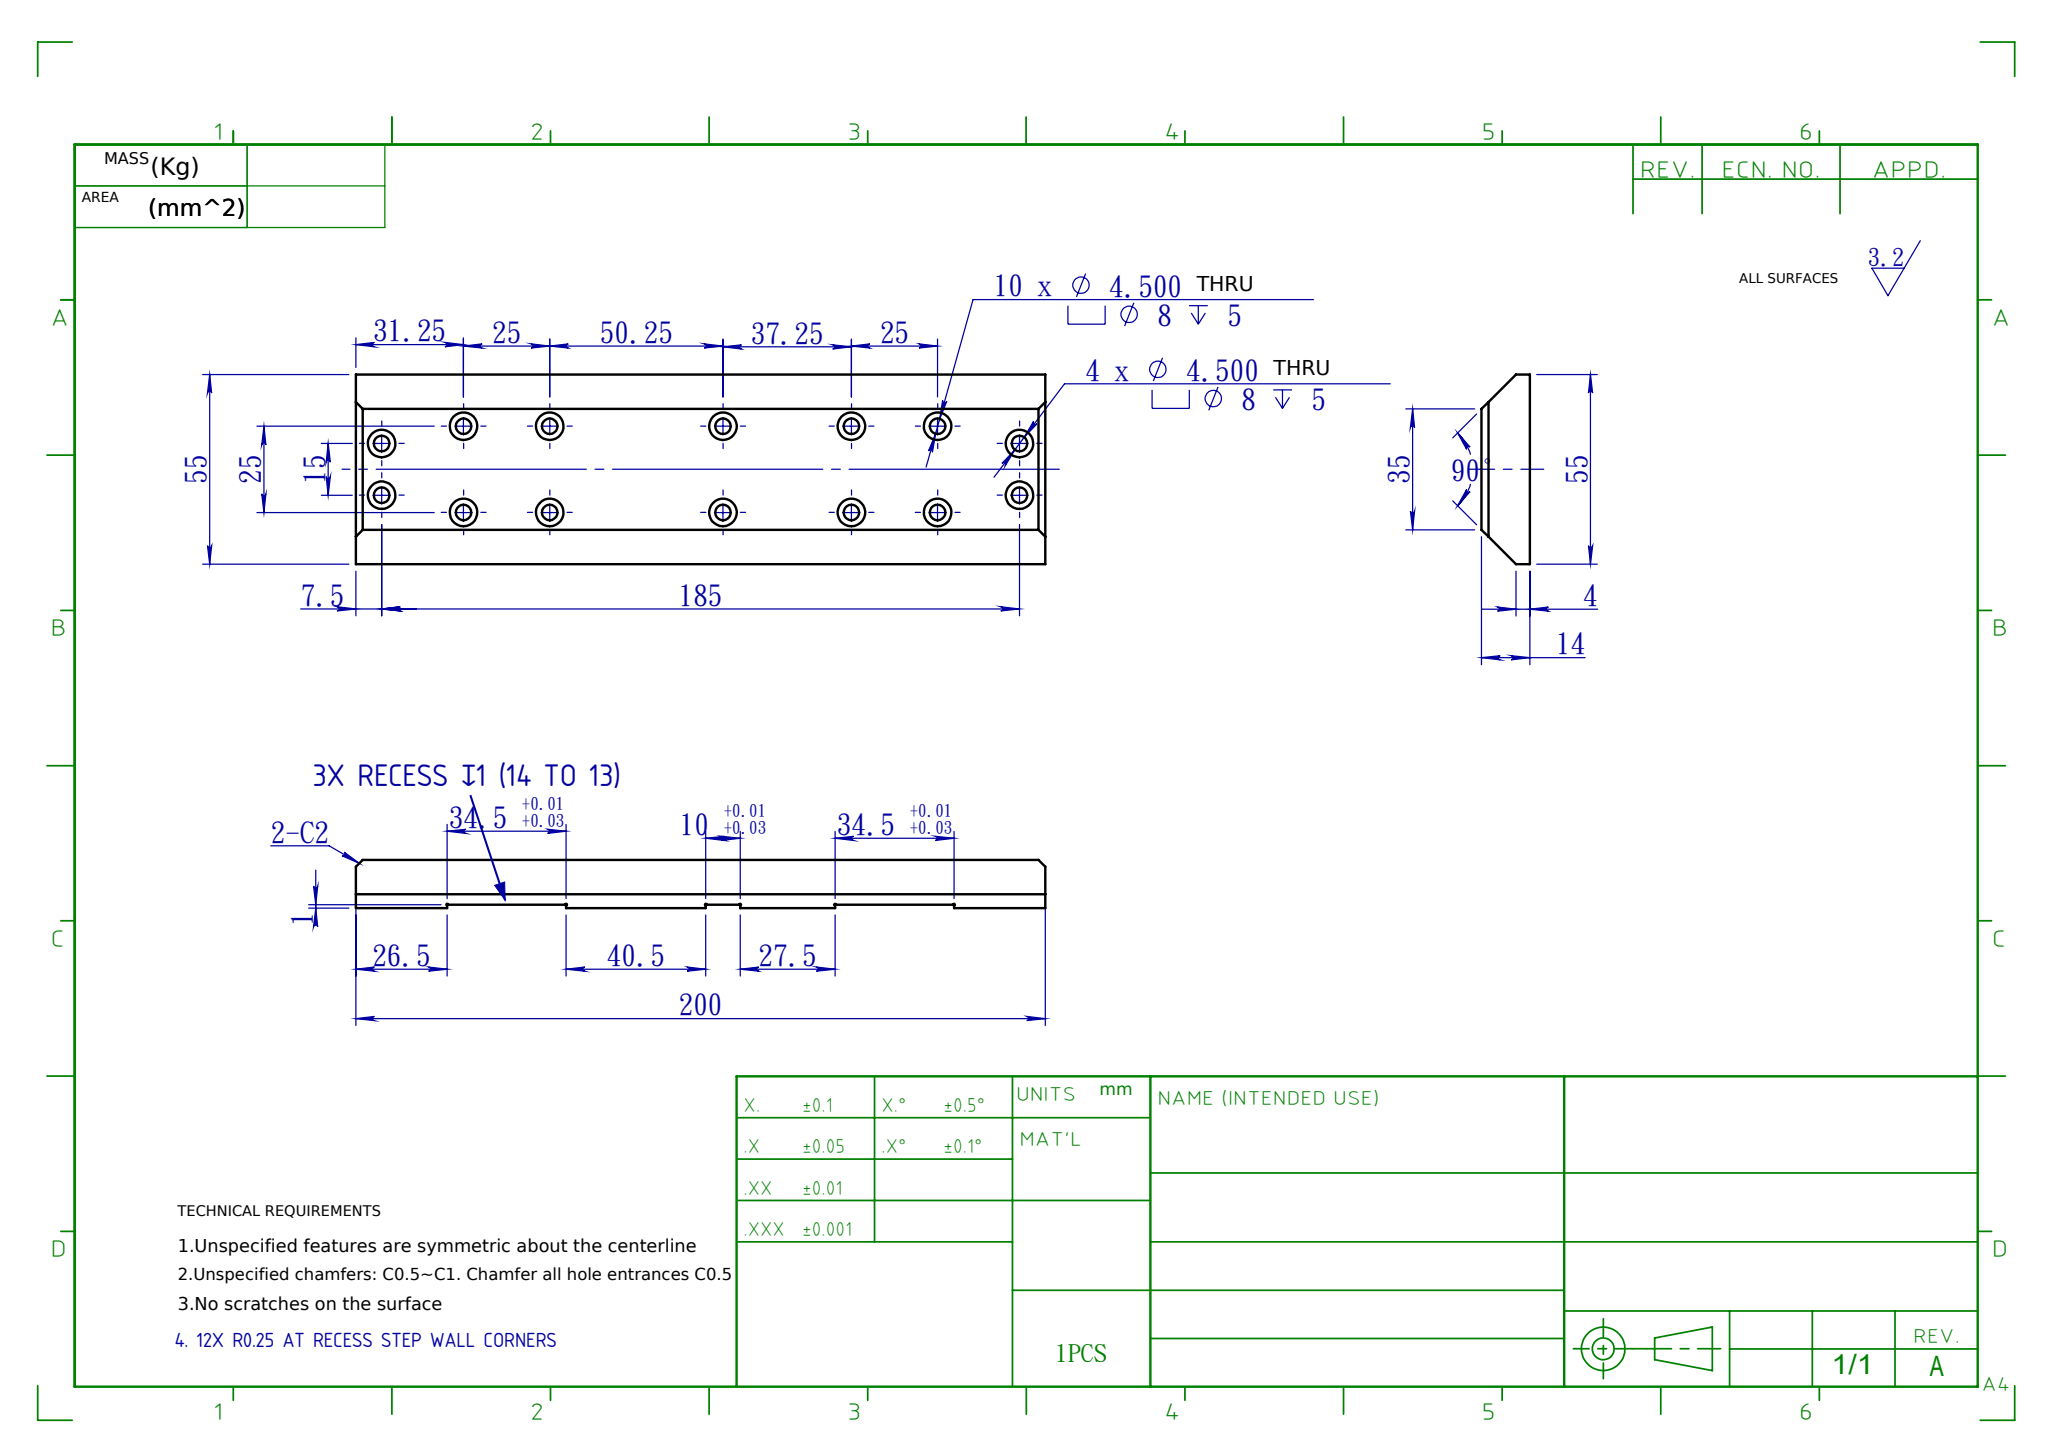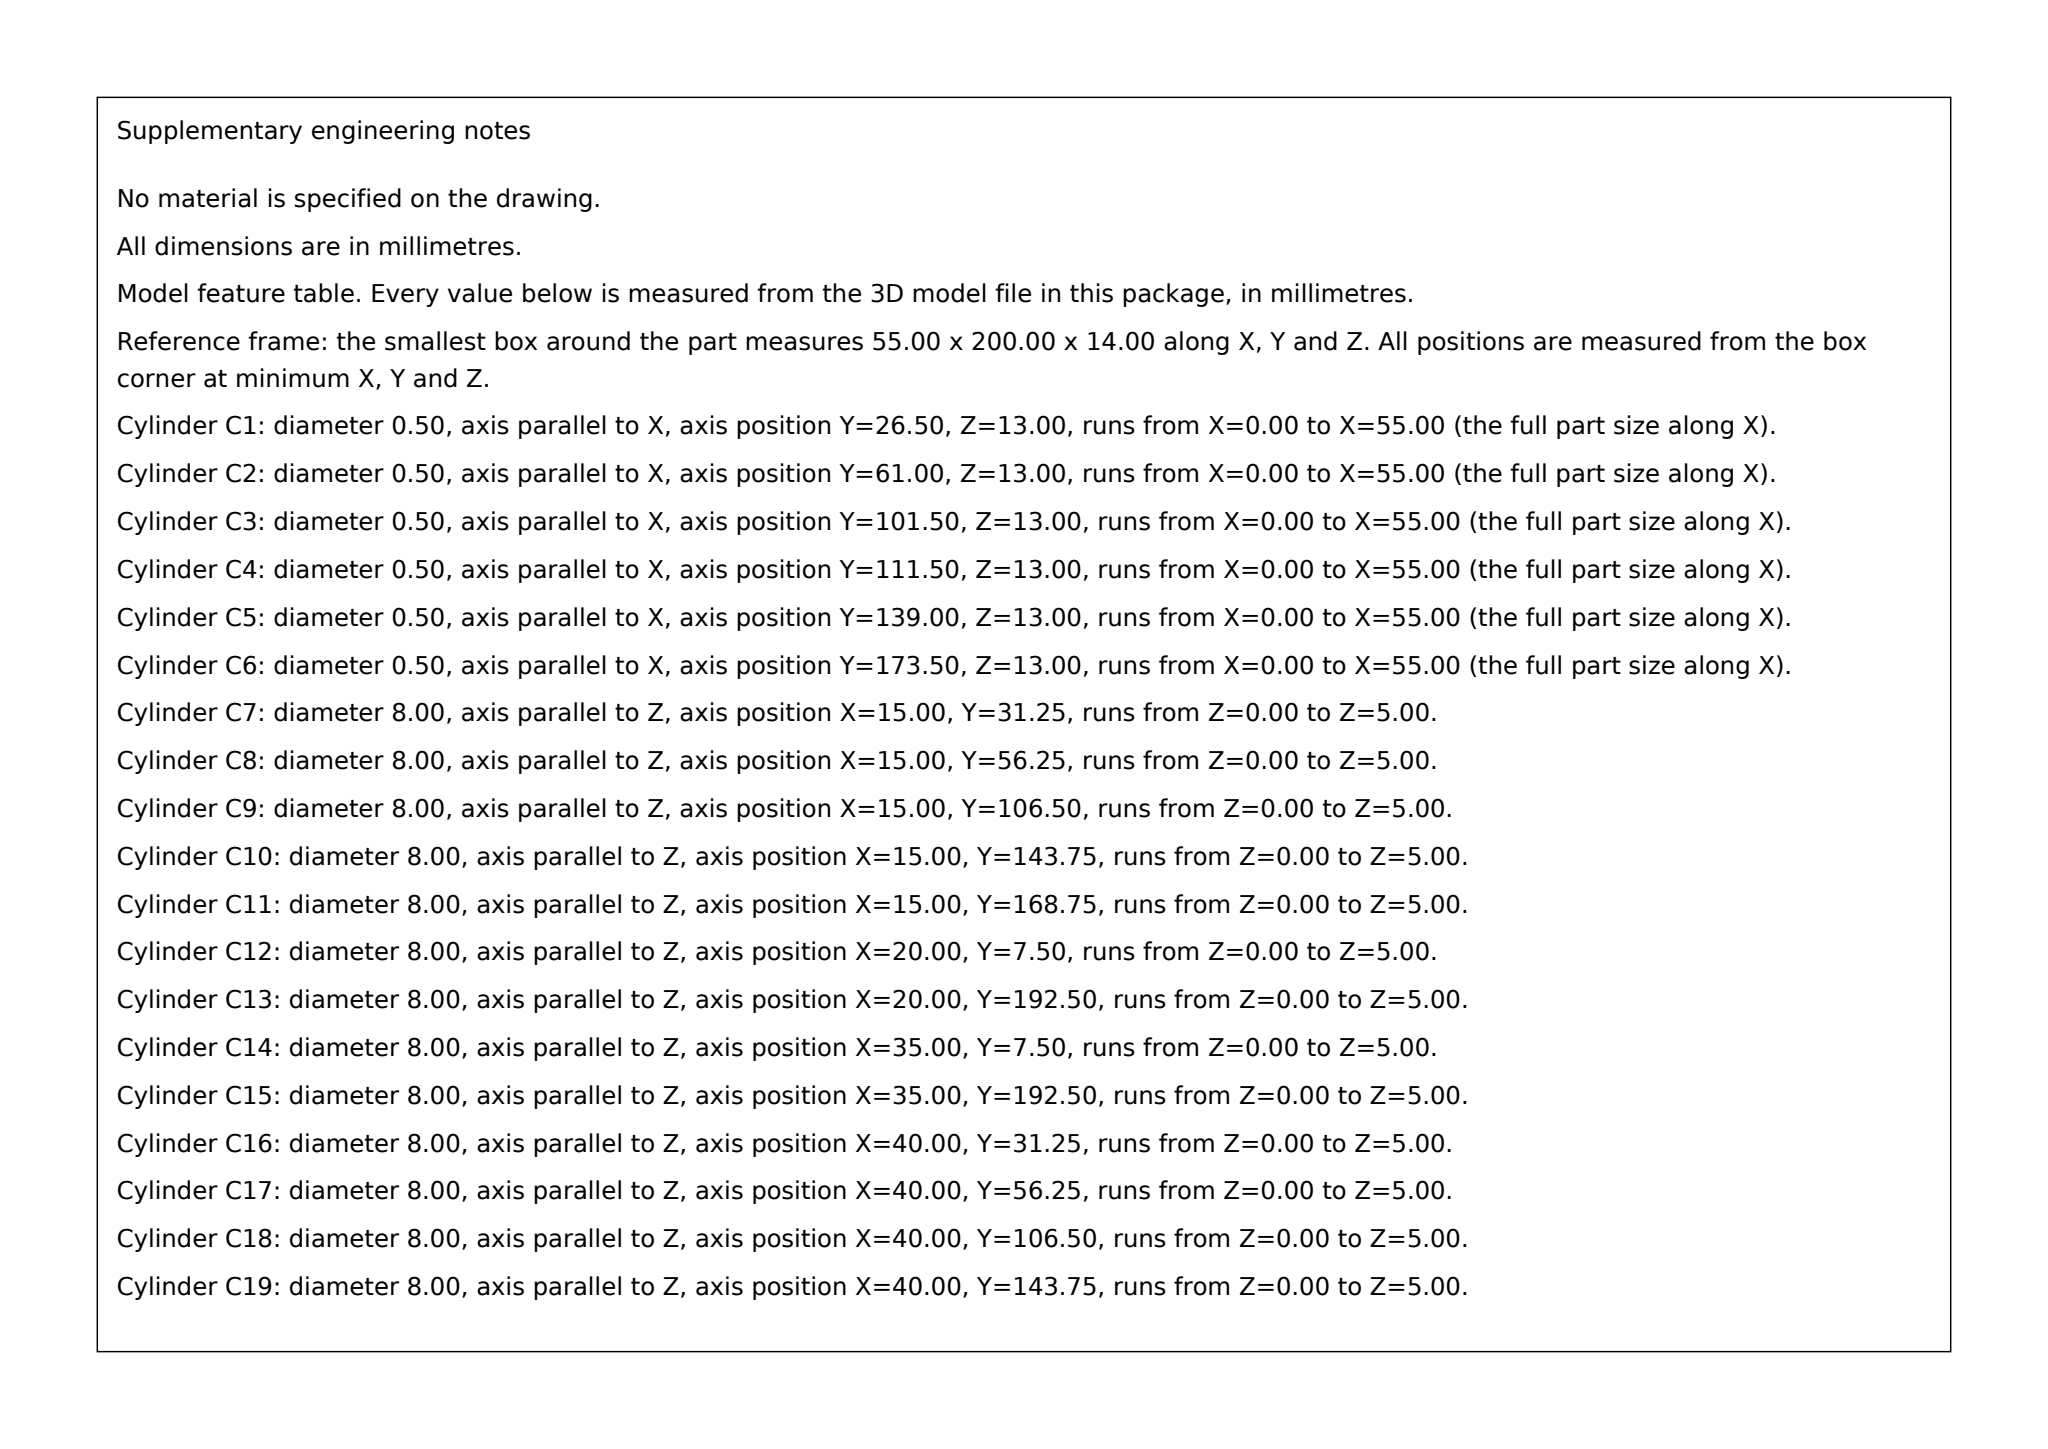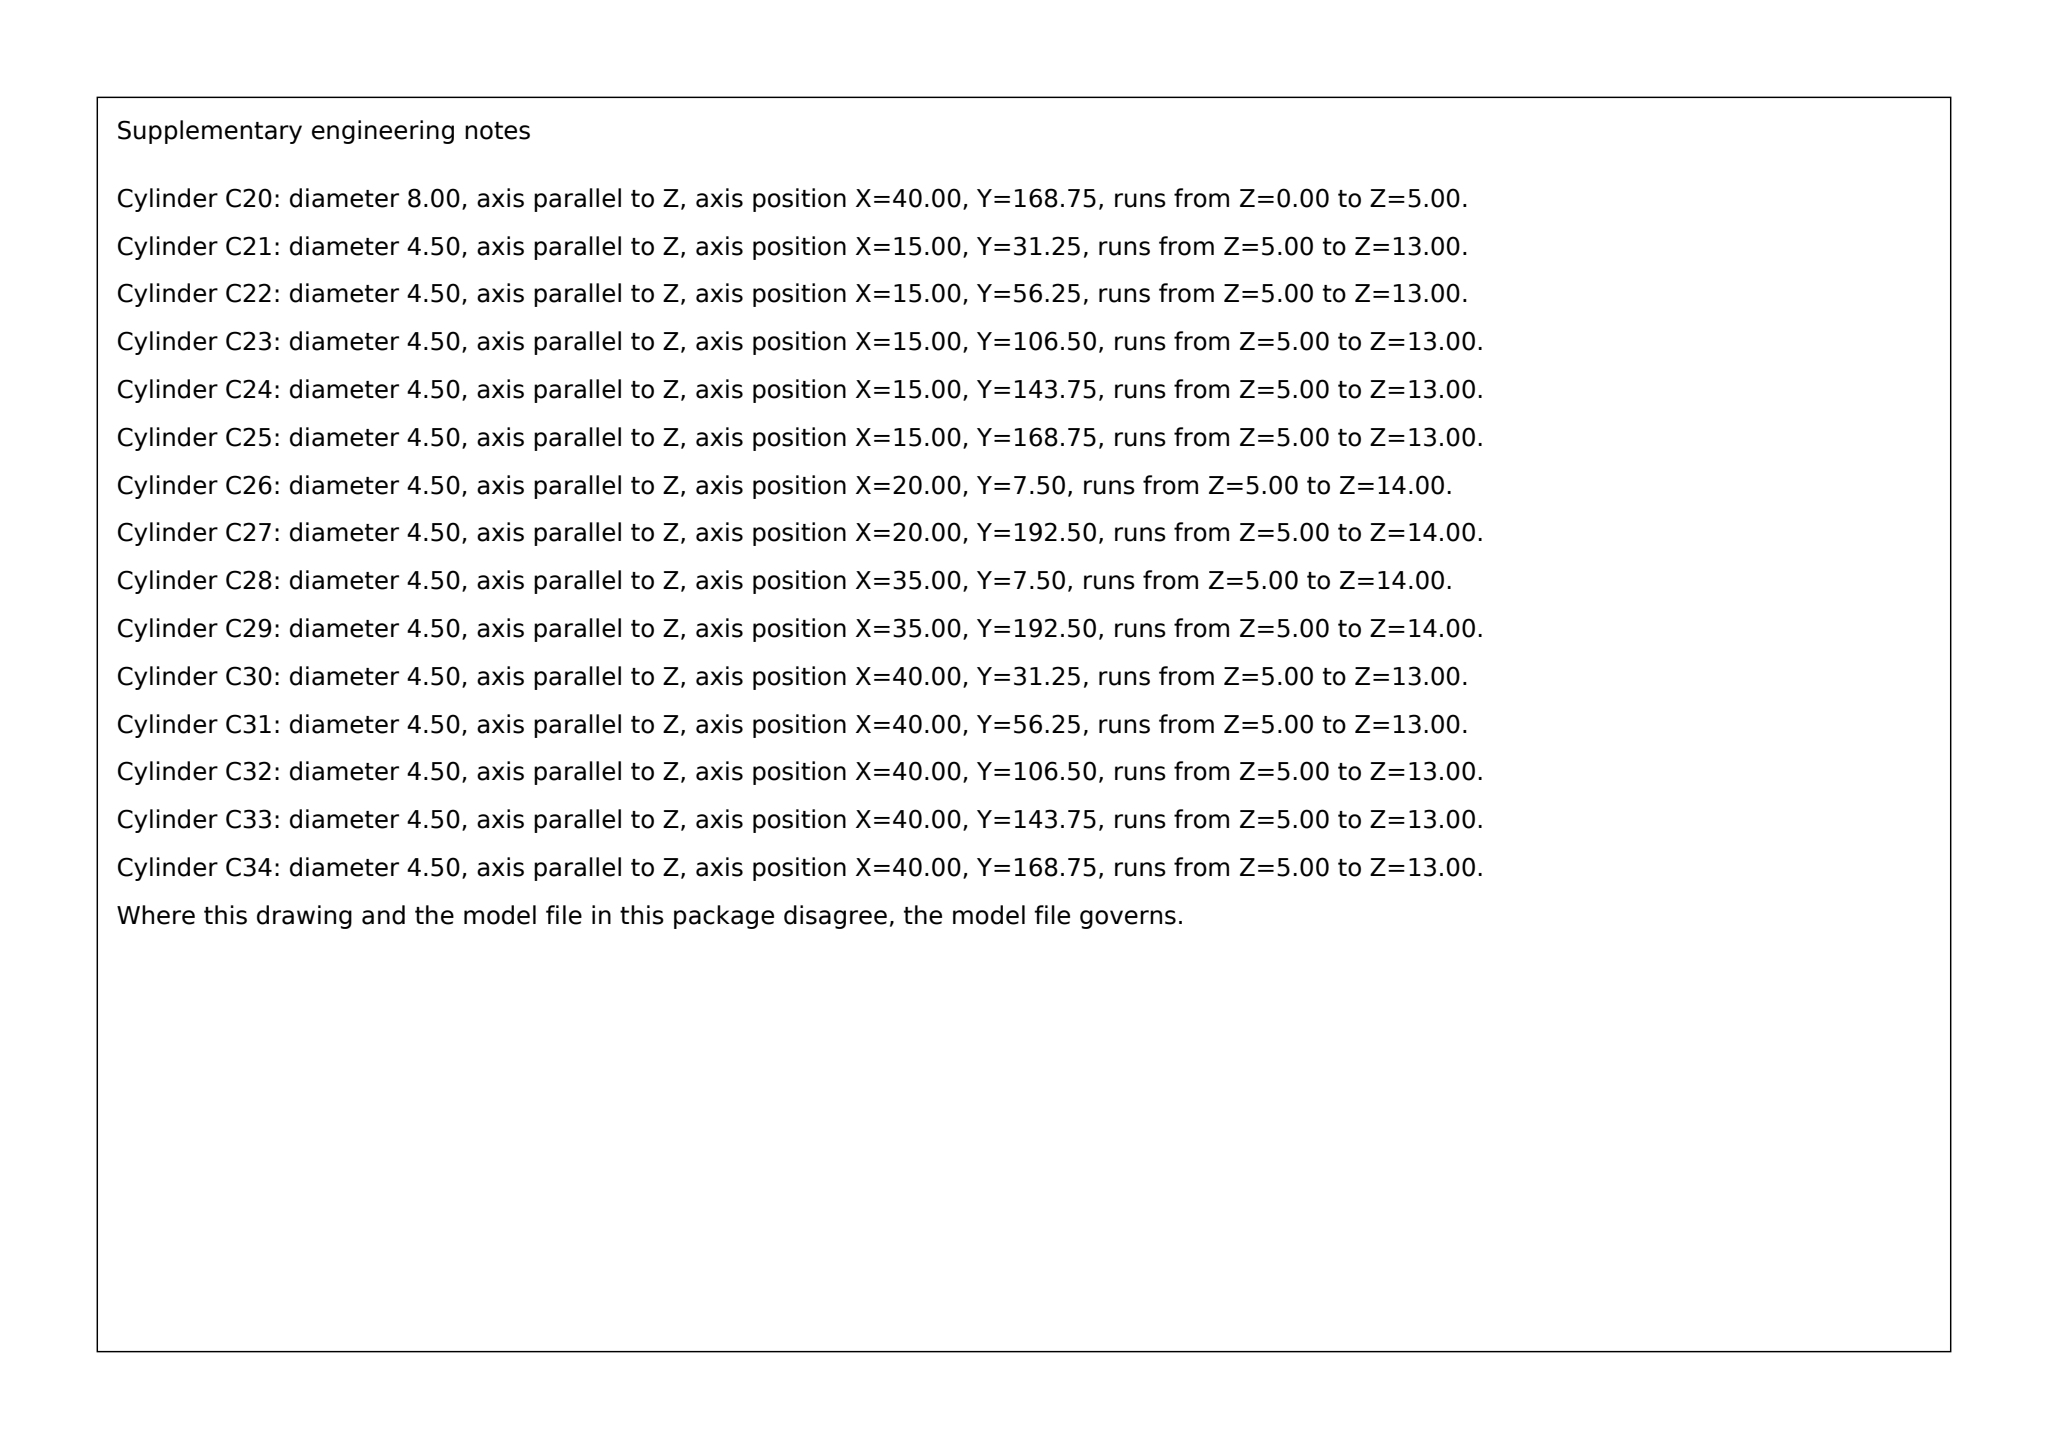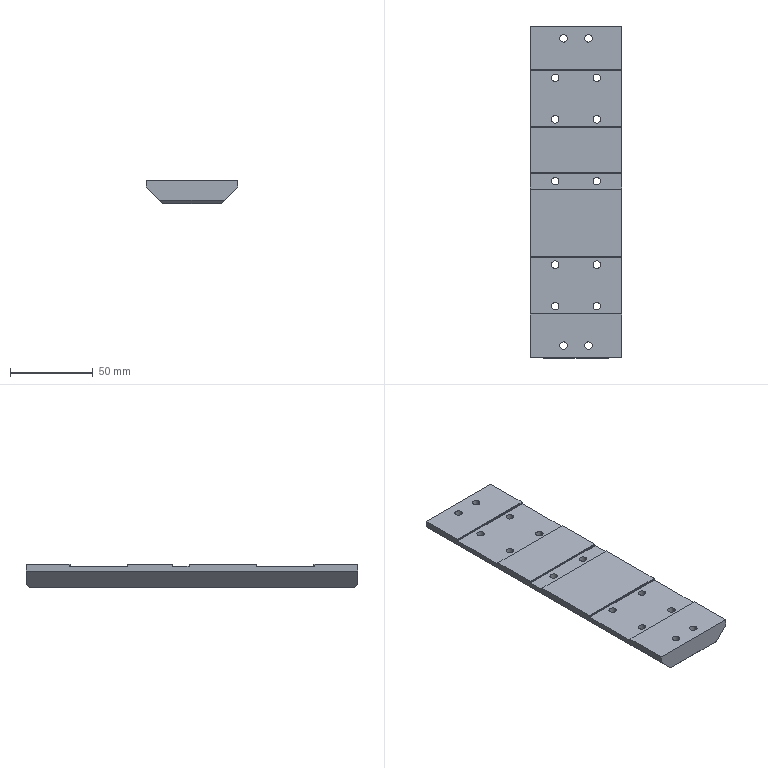Part | SolidWorks | mm | 1 solid | 104 faces | box 55 x 200 x 14 mm | volume 124098 mm3 | cylinder 68 | plane 36 | commonest cylinder face diameters 8 x28 4.5 x28 0.5 x12
Drawing notes:
3X RECESS IN 35 TOP FACE: 1 DEEP (14 TO 13 OAH) | from the solid: z-planes at 14.0 (top) and 13.0 (3 recess floors); bbox Z=14
12X R0.25 AT RECESS STEP WALL CORNERS | from the solid: Ø0.5 x-axis cylinders at z=13.0, y=26.5/61/101.5/111.5/139/173.5, 2 each
build123d program:
from build123d import *

# Parameters (mm, degrees)
SKETCH1_2_W                                         = 55
SKETCH1_2_H                                         = 200
BOSS_EXTRUDE1_DEPTH                                 = 14
SKETCH2_2_W                                         = 55
SKETCH2_2_H                                         = 34.5
SKETCH2_2_H_2                                       = 10
BOSS_EXTRUDE2_DEPTH                                 = 20
CHAMFER1_SIZE                                       = 10
SKETCH3_2_W                                         = 55
SKETCH3_2_H                                         = 20
CUT_EXTRUDE1_2_DEPTH                                = 15
CBORE_FOR_M4_HEX_SOCKET_HEAD_CAP_SCREW1_D           = 4.5
CBORE_FOR_M4_HEX_SOCKET_HEAD_CAP_SCREW1_CBORE_D     = 8
CBORE_FOR_M4_HEX_SOCKET_HEAD_CAP_SCREW1_CBORE_DEPTH = 5
M4_TAPPED_HOLE1_D                                   = 3.3
SKETCH11_W                                          = 21
SKETCH11_H                                          = 34.5
SKETCH11_H_2                                        = 10
CUT_EXTRUDE2_DEPTH                                  = 120.084
CHAMFER2_SIZE                                       = 2
CBORE_FOR_M4_HEX_SOCKET_HEAD_CAP_SCREW2_D           = 4.5
CBORE_FOR_M4_HEX_SOCKET_HEAD_CAP_SCREW2_CBORE_D     = 8
CBORE_FOR_M4_HEX_SOCKET_HEAD_CAP_SCREW2_CBORE_DEPTH = 5
SKETCH3_R                                           = 0.25
CUT_EXTRUDE1_DEPTH                                  = 115.983


with BuildPart() as part:
    # Sketch1_2 → Boss-Extrude1 (new body)
    with BuildSketch(Plane.XY):
        Rectangle(SKETCH1_2_W, SKETCH1_2_H)
    extrude(amount=BOSS_EXTRUDE1_DEPTH)

    # Sketch2_2 → Boss-Extrude2 (add)
    with BuildSketch(Plane.XY.offset(14)):
        with Locations((0, 56.25)):
            Rectangle(SKETCH2_2_W, SKETCH2_2_H)
        with Locations((0, 6.5)):
            Rectangle(SKETCH2_2_W, SKETCH2_2_H_2)
        with Locations((0, -56.25)):
            Rectangle(SKETCH2_2_W, SKETCH2_2_H)
    extrude(amount=BOSS_EXTRUDE2_DEPTH)

    # Chamfer1
    chamfer1_edges = [part.edges().sort_by_distance(p)[0] for p in [
        (27.5, 0, 0),
        (-27.5, 0, 0),
    ]]
    chamfer(chamfer1_edges, length=CHAMFER1_SIZE)

    # Sketch3_2 → Cut-Extrude1_2 (cut)
    with BuildSketch(Plane.XY.offset(34)):
        with Locations((0, 56.25)):
            Rectangle(SKETCH3_2_W, SKETCH3_2_H)
        with Locations((0, -56.25)):
            Rectangle(SKETCH3_2_W, SKETCH3_2_H)
    extrude(amount=-CUT_EXTRUDE1_2_DEPTH, mode=Mode.SUBTRACT)

    # CBORE for M4 Hex Socket Head Cap Screw1 (through all)
    with Locations(Plane(origin=(0, 0, 0), x_dir=(-1, 0, 0), z_dir=(0, 0, -1))):
        with Locations((7.5, -92.5), (-7.5, -92.5), (7.5, 92.5), (-7.5, 92.5)):
            CounterBoreHole(CBORE_FOR_M4_HEX_SOCKET_HEAD_CAP_SCREW1_D / 2, CBORE_FOR_M4_HEX_SOCKET_HEAD_CAP_SCREW1_CBORE_D / 2, CBORE_FOR_M4_HEX_SOCKET_HEAD_CAP_SCREW1_CBORE_DEPTH)

    # M4 Tapped Hole1 (through all)
    with Locations(Plane(origin=(0, 73.5, 0), x_dir=(1, 0, 0), z_dir=(0, 1, 0))):
        with Locations((-15, -27.5), (15, -27.5)):
            Hole(M4_TAPPED_HOLE1_D / 2)

    # Sketch11 → Cut-Extrude2 (cut, through all)
    with BuildSketch(Plane(origin=(27.5, 0, 0), x_dir=(0, 0, -1), z_dir=(1, 0, 0))):
        with Locations((-23.5, 56.25)):
            Rectangle(SKETCH11_W, SKETCH11_H)
        with Locations((-23.5, 6.5)):
            Rectangle(SKETCH11_W, SKETCH11_H_2)
        with Locations((-23.5, -56.25)):
            Rectangle(SKETCH11_W, SKETCH11_H)
    extrude(amount=-CUT_EXTRUDE2_DEPTH, mode=Mode.SUBTRACT)

    # Chamfer2
    chamfer2_edges = [part.edges().sort_by_distance(p)[0] for p in [
        (0, -100, 0),
        (0, 100, 0),
    ]]
    chamfer(chamfer2_edges, length=CHAMFER2_SIZE)

    # CBORE for M4 Hex Socket Head Cap Screw2 (through all)
    with Locations(Plane(origin=(0, 0, 0), x_dir=(-1, 0, 0), z_dir=(0, 0, -1))):
        with Locations((-12.5, 68.75), (12.5, 68.75), (-12.5, 43.75), (12.5, 43.75), (-12.5, 6.5), (12.5, 6.5), (-12.5, -43.75), (12.5, -43.75), (-12.5, -68.75), (12.5, -68.75)):
            CounterBoreHole(CBORE_FOR_M4_HEX_SOCKET_HEAD_CAP_SCREW2_D / 2, CBORE_FOR_M4_HEX_SOCKET_HEAD_CAP_SCREW2_CBORE_D / 2, CBORE_FOR_M4_HEX_SOCKET_HEAD_CAP_SCREW2_CBORE_DEPTH)

    # Sketch3 → Cut-Extrude1 (cut, through all)
    with BuildSketch(Plane(origin=(27.5, 0, 0), x_dir=(0, 0, -1), z_dir=(1, 0, 0))):
        with Locations((-13, 73.5)):
            Circle(SKETCH3_R)
        with Locations((-13, 39)):
            Circle(SKETCH3_R)
        with Locations((-13, 11.5)):
            Circle(SKETCH3_R)
        with Locations((-13, 1.5)):
            Circle(SKETCH3_R)
        with Locations((-13, -39)):
            Circle(SKETCH3_R)
        with Locations((-13, -73.5)):
            Circle(SKETCH3_R)
    extrude(amount=-CUT_EXTRUDE1_DEPTH, mode=Mode.SUBTRACT)


solid = part.part